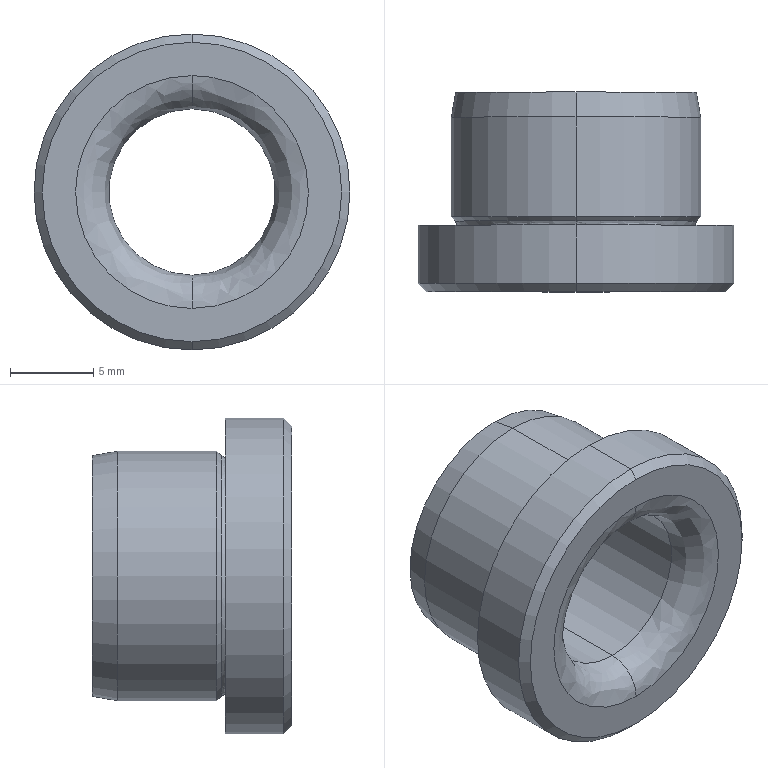Component | SolidWorks | JBH10-8-1 | 1 solid | 21 faces | box 19 x 12 x 19 mm | volume 1544 mm3 | cone 8 | cylinder 6 | spline 4 | plane 3 | commonest cylinder face diameters 10 x2 15 x2 19 x2 | material '-
STEP:
#1=COLOUR_RGB('',0.7922,0.8196,0.9333);
#2=FILL_AREA_STYLE_COLOUR('',#1);
#3=FILL_AREA_STYLE('',(#2));
#4=SURFACE_STYLE_FILL_AREA(#3);
#5=SURFACE_SIDE_STYLE('',(#4));
#6=SURFACE_STYLE_USAGE(.BOTH.,#5);
#7=PRESENTATION_STYLE_ASSIGNMENT((#6));
#8=CARTESIAN_POINT('',(-1.614,3.16,0.1969));
#9=VERTEX_POINT('',#8);
#10=CARTESIAN_POINT('',(-1.614,3.16,-0.1969));
#11=VERTEX_POINT('',#10);
#12=CARTESIAN_POINT('',(-1.614,3.16,-0.));
#13=DIRECTION('',(0.,1.,0.));
#14=DIRECTION('',(0.,0.,-1.));
#15=AXIS2_PLACEMENT_3D('',#12,#13,#14);
#16=CIRCLE('',#15,0.1969);
#17=EDGE_CURVE('',#9,#11,#16,.T.);
#18=ORIENTED_EDGE('',*,*,#17,.T.);
#19=CARTESIAN_POINT('',(-1.614,3.081,-0.2756));
#20=VERTEX_POINT('',#19);
#21=CARTESIAN_POINT('',(-1.614,3.16,-0.2756));
#22=DIRECTION('',(1.,0.,-0.));
#23=DIRECTION('',(0.,0.,-1.));
#24=AXIS2_PLACEMENT_3D('',#21,#22,#23);
#25=CIRCLE('',#24,0.07874);
#26=EDGE_CURVE('',#11,#20,#25,.T.);
#27=ORIENTED_EDGE('',*,*,#26,.T.);
#28=CARTESIAN_POINT('',(-1.614,3.081,0.2756));
#29=VERTEX_POINT('',#28);
#30=CARTESIAN_POINT('',(-1.614,3.081,-0.2756));
#31=CARTESIAN_POINT('',(-1.063,3.081,-0.2756));
#32=CARTESIAN_POINT('',(-1.063,3.081,0.2756));
#33=CARTESIAN_POINT('',(-1.614,3.081,0.2756));
#34=(BOUNDED_CURVE()B_SPLINE_CURVE(3,(#30,#31,#32,#33),.UNSPECIFIED.,.F.,.F.)B_SPLINE_CURVE_WITH_KNOTS((4,4),(0.,1.),.UNSPECIFIED.)CURVE()GEOMETRIC_REPRESENTATION_ITEM()RATIONAL_B_SPLINE_CURVE((1.,0.3333,0.3333,1.))REPRESENTATION_ITEM(''));
#35=EDGE_CURVE('',#20,#29,#34,.T.);
#36=ORIENTED_EDGE('',*,*,#35,.T.);
#37=CARTESIAN_POINT('',(-1.614,3.16,0.2756));
#38=DIRECTION('',(-1.,0.,0.));
#39=DIRECTION('',(0.,0.,1.));
#40=AXIS2_PLACEMENT_3D('',#37,#38,#39);
#41=CIRCLE('',#40,0.07874);
#42=EDGE_CURVE('',#9,#29,#41,.T.);
#43=ORIENTED_EDGE('',*,*,#42,.F.);
#44=EDGE_LOOP('',(#18,#27,#36,#43));
#45=FACE_OUTER_BOUND('',#44,.T.);
#46=CARTESIAN_POINT('',(-1.614,3.16,-0.1969));
#47=CARTESIAN_POINT('',(-1.22,3.16,-0.1969));
#48=CARTESIAN_POINT('',(-1.22,3.16,0.1969));
#49=CARTESIAN_POINT('',(-1.614,3.16,0.1969));
#50=CARTESIAN_POINT('',(-1.614,3.113,-0.1969));
#51=CARTESIAN_POINT('',(-1.22,3.113,-0.1969));
#52=CARTESIAN_POINT('',(-1.22,3.113,0.1969));
#53=CARTESIAN_POINT('',(-1.614,3.113,0.1969));
#54=CARTESIAN_POINT('',(-1.614,3.081,-0.2295));
#55=CARTESIAN_POINT('',(-1.155,3.081,-0.2295));
#56=CARTESIAN_POINT('',(-1.155,3.081,0.2295));
#57=CARTESIAN_POINT('',(-1.614,3.081,0.2295));
#58=CARTESIAN_POINT('',(-1.614,3.081,-0.2756));
#59=CARTESIAN_POINT('',(-1.063,3.081,-0.2756));
#60=CARTESIAN_POINT('',(-1.063,3.081,0.2756));
#61=CARTESIAN_POINT('',(-1.614,3.081,0.2756));
#62=(BOUNDED_SURFACE()B_SPLINE_SURFACE(3,3,((#46,#47,#48,#49),(#50,#51,#52,#53),(#54,#55,#56,#57),(#58,#59,#60,#61)),.UNSPECIFIED.,.F.,.F.,.T.)B_SPLINE_SURFACE_WITH_KNOTS((4,4),(4,4),(0.,1.),(0.,1.),.UNSPECIFIED.)GEOMETRIC_REPRESENTATION_ITEM()RATIONAL_B_SPLINE_SURFACE(((1.,0.3333,0.3333,1.),(0.8047,0.2682,0.2682,0.8047),(0.8047,0.2682,0.2682,0.8047),(1.,0.3333,0.3333,1.)))REPRESENTATION_ITEM('')SURFACE());
#63=ADVANCED_FACE('',(#45),#62,.T.);
#64=CARTESIAN_POINT('',(-1.614,3.248,-0.2854));
#65=VERTEX_POINT('',#64);
#66=CARTESIAN_POINT('',(-1.614,3.248,0.2854));
#67=VERTEX_POINT('',#66);
#68=CARTESIAN_POINT('',(-1.614,3.248,-0.));
#69=DIRECTION('',(0.,1.,0.));
#70=DIRECTION('',(-1.,0.,-0.));
#71=AXIS2_PLACEMENT_3D('',#68,#69,#70);
#72=CIRCLE('',#71,0.2854);
#73=EDGE_CURVE('',#65,#67,#72,.T.);
#74=ORIENTED_EDGE('',*,*,#73,.F.);
#75=CARTESIAN_POINT('',(-1.614,3.228,-0.3051));
#76=VERTEX_POINT('',#75);
#77=CARTESIAN_POINT('',(-1.614,3.238,-0.2953));
#78=DIRECTION('',(1.,0.,-0.));
#79=DIRECTION('',(0.,0.,-1.));
#80=AXIS2_PLACEMENT_3D('',#77,#78,#79);
#81=CIRCLE('',#80,0.01392);
#82=EDGE_CURVE('',#65,#76,#81,.T.);
#83=ORIENTED_EDGE('',*,*,#82,.T.);
#84=CARTESIAN_POINT('',(-1.614,3.228,0.3051));
#85=VERTEX_POINT('',#84);
#86=CARTESIAN_POINT('',(-1.614,3.228,-0.));
#87=DIRECTION('',(0.,-1.,0.));
#88=DIRECTION('',(0.,0.,1.));
#89=AXIS2_PLACEMENT_3D('',#86,#87,#88);
#90=CIRCLE('',#89,0.3051);
#91=EDGE_CURVE('',#85,#76,#90,.T.);
#92=ORIENTED_EDGE('',*,*,#91,.F.);
#93=CARTESIAN_POINT('',(-1.614,3.238,0.2953));
#94=DIRECTION('',(-1.,0.,0.));
#95=DIRECTION('',(0.,0.,1.));
#96=AXIS2_PLACEMENT_3D('',#93,#94,#95);
#97=CIRCLE('',#96,0.01392);
#98=EDGE_CURVE('',#67,#85,#97,.T.);
#99=ORIENTED_EDGE('',*,*,#98,.F.);
#100=EDGE_LOOP('',(#74,#83,#92,#99));
#101=FACE_OUTER_BOUND('',#100,.T.);
#102=CARTESIAN_POINT('',(-1.614,3.248,0.2854));
#103=CARTESIAN_POINT('',(-2.185,3.248,0.2854));
#104=CARTESIAN_POINT('',(-2.185,3.248,-0.2854));
#105=CARTESIAN_POINT('',(-1.614,3.248,-0.2854));
#106=CARTESIAN_POINT('',(-1.614,3.242,0.2797));
#107=CARTESIAN_POINT('',(-2.174,3.242,0.2797));
#108=CARTESIAN_POINT('',(-2.174,3.242,-0.2797));
#109=CARTESIAN_POINT('',(-1.614,3.242,-0.2797));
#110=CARTESIAN_POINT('',(-1.614,3.234,0.2797));
#111=CARTESIAN_POINT('',(-2.174,3.234,0.2797));
#112=CARTESIAN_POINT('',(-2.174,3.234,-0.2797));
#113=CARTESIAN_POINT('',(-1.614,3.234,-0.2797));
#114=CARTESIAN_POINT('',(-1.614,3.228,0.2854));
#115=CARTESIAN_POINT('',(-2.185,3.228,0.2854));
#116=CARTESIAN_POINT('',(-2.185,3.228,-0.2854));
#117=CARTESIAN_POINT('',(-1.614,3.228,-0.2854));
#118=CARTESIAN_POINT('',(-1.614,3.223,0.2912));
#119=CARTESIAN_POINT('',(-2.197,3.223,0.2912));
#120=CARTESIAN_POINT('',(-2.197,3.223,-0.2912));
#121=CARTESIAN_POINT('',(-1.614,3.223,-0.2912));
#122=CARTESIAN_POINT('',(-1.614,3.223,0.2994));
#123=CARTESIAN_POINT('',(-2.213,3.223,0.2994));
#124=CARTESIAN_POINT('',(-2.213,3.223,-0.2994));
#125=CARTESIAN_POINT('',(-1.614,3.223,-0.2994));
#126=CARTESIAN_POINT('',(-1.614,3.228,0.3051));
#127=CARTESIAN_POINT('',(-2.224,3.228,0.3051));
#128=CARTESIAN_POINT('',(-2.224,3.228,-0.3051));
#129=CARTESIAN_POINT('',(-1.614,3.228,-0.3051));
#130=(BOUNDED_SURFACE()B_SPLINE_SURFACE(3,3,((#102,#103,#104,#105),(#106,#107,#108,#109),(#110,#111,#112,#113),(#114,#115,#116,#117),(#118,#119,#120,#121),(#122,#123,#124,#125),(#126,#127,#128,#129)),.UNSPECIFIED.,.F.,.F.,.T.)B_SPLINE_SURFACE_WITH_KNOTS((4,3,4),(4,4),(0.,0.5,1.),(0.,1.),.UNSPECIFIED.)GEOMETRIC_REPRESENTATION_ITEM()RATIONAL_B_SPLINE_SURFACE(((1.,0.3333,0.3333,1.),(0.8047,0.2682,0.2682,0.8047),(0.8047,0.2682,0.2682,0.8047),(1.,0.3333,0.3333,1.),(0.8047,0.2682,0.2682,0.8047),(0.8047,0.2682,0.2682,0.8047),(1.,0.3333,0.3333,1.)))REPRESENTATION_ITEM('')SURFACE());
#131=ADVANCED_FACE('',(#101),#130,.F.);
#132=ORIENTED_EDGE('',*,*,#17,.F.);
#133=CARTESIAN_POINT('',(-1.614,3.553,0.1969));
#134=VERTEX_POINT('',#133);
#135=CARTESIAN_POINT('',(-1.614,3.356,0.1969));
#136=DIRECTION('',(0.,1.,0.));
#137=VECTOR('',#136,39.37);
#138=LINE('',#135,#137);
#139=EDGE_CURVE('',#9,#134,#138,.T.);
#140=ORIENTED_EDGE('',*,*,#139,.T.);
#141=CARTESIAN_POINT('',(-1.614,3.553,-0.1969));
#142=VERTEX_POINT('',#141);
#143=CARTESIAN_POINT('',(-1.614,3.553,-0.));
#144=DIRECTION('',(0.,-1.,0.));
#145=DIRECTION('',(0.,0.,-1.));
#146=AXIS2_PLACEMENT_3D('',#143,#144,#145);
#147=CIRCLE('',#146,0.1969);
#148=EDGE_CURVE('',#142,#134,#147,.T.);
#149=ORIENTED_EDGE('',*,*,#148,.F.);
#150=CARTESIAN_POINT('',(-1.614,3.356,-0.1969));
#151=DIRECTION('',(0.,1.,0.));
#152=VECTOR('',#151,39.37);
#153=LINE('',#150,#152);
#154=EDGE_CURVE('',#11,#142,#153,.T.);
#155=ORIENTED_EDGE('',*,*,#154,.F.);
#156=EDGE_LOOP('',(#132,#140,#149,#155));
#157=FACE_OUTER_BOUND('',#156,.T.);
#158=CARTESIAN_POINT('',(-1.614,3.356,-0.));
#159=DIRECTION('',(0.,1.,0.));
#160=DIRECTION('',(0.,0.,-1.));
#161=AXIS2_PLACEMENT_3D('',#158,#159,#160);
#162=CYLINDRICAL_SURFACE('',#161,0.1969);
#163=ADVANCED_FACE('',(#157),#162,.F.);
#164=CARTESIAN_POINT('',(-1.614,3.553,-0.2849));
#165=VERTEX_POINT('',#164);
#166=CARTESIAN_POINT('',(-1.614,3.553,0.2849));
#167=VERTEX_POINT('',#166);
#168=CARTESIAN_POINT('',(-1.614,3.553,-0.));
#169=DIRECTION('',(0.,1.,0.));
#170=DIRECTION('',(0.,0.,1.));
#171=AXIS2_PLACEMENT_3D('',#168,#169,#170);
#172=CIRCLE('',#171,0.2849);
#173=EDGE_CURVE('',#165,#167,#172,.T.);
#174=ORIENTED_EDGE('',*,*,#173,.F.);
#175=CARTESIAN_POINT('',(-1.614,3.494,-0.2953));
#176=VERTEX_POINT('',#175);
#177=CARTESIAN_POINT('',(-1.614,3.494,-0.2953));
#178=DIRECTION('',(-0.,-0.9848,-0.1736));
#179=VECTOR('',#178,39.37);
#180=LINE('',#177,#179);
#181=EDGE_CURVE('',#165,#176,#180,.T.);
#182=ORIENTED_EDGE('',*,*,#181,.T.);
#183=CARTESIAN_POINT('',(-1.614,3.494,0.2953));
#184=VERTEX_POINT('',#183);
#185=CARTESIAN_POINT('',(-1.614,3.494,-0.));
#186=DIRECTION('',(0.,1.,0.));
#187=DIRECTION('',(-1.,0.,-0.));
#188=AXIS2_PLACEMENT_3D('',#185,#186,#187);
#189=CIRCLE('',#188,0.2953);
#190=EDGE_CURVE('',#176,#184,#189,.T.);
#191=ORIENTED_EDGE('',*,*,#190,.T.);
#192=CARTESIAN_POINT('',(-1.614,3.494,0.2953));
#193=DIRECTION('',(0.,-0.9848,0.1736));
#194=VECTOR('',#193,39.37);
#195=LINE('',#192,#194);
#196=EDGE_CURVE('',#167,#184,#195,.T.);
#197=ORIENTED_EDGE('',*,*,#196,.F.);
#198=EDGE_LOOP('',(#174,#182,#191,#197));
#199=FACE_OUTER_BOUND('',#198,.T.);
#200=CARTESIAN_POINT('',(-1.614,3.494,-0.));
#201=DIRECTION('',(0.,-1.,0.));
#202=DIRECTION('',(0.,0.,1.));
#203=AXIS2_PLACEMENT_3D('',#200,#201,#202);
#204=CONICAL_SURFACE('',#203,0.2953,0.1745);
#205=ADVANCED_FACE('',(#199),#204,.T.);
#206=CARTESIAN_POINT('',(-1.614,3.258,-0.2953));
#207=VERTEX_POINT('',#206);
#208=CARTESIAN_POINT('',(-1.614,3.258,0.2953));
#209=VERTEX_POINT('',#208);
#210=CARTESIAN_POINT('',(-1.614,3.258,-0.));
#211=DIRECTION('',(0.,1.,0.));
#212=DIRECTION('',(0.,0.,-1.));
#213=AXIS2_PLACEMENT_3D('',#210,#211,#212);
#214=CIRCLE('',#213,0.2953);
#215=EDGE_CURVE('',#207,#209,#214,.T.);
#216=ORIENTED_EDGE('',*,*,#215,.T.);
#217=CARTESIAN_POINT('',(-1.614,3.376,0.2953));
#218=DIRECTION('',(0.,1.,0.));
#219=VECTOR('',#218,39.37);
#220=LINE('',#217,#219);
#221=EDGE_CURVE('',#209,#184,#220,.T.);
#222=ORIENTED_EDGE('',*,*,#221,.T.);
#223=ORIENTED_EDGE('',*,*,#190,.F.);
#224=CARTESIAN_POINT('',(-1.614,3.376,-0.2953));
#225=DIRECTION('',(0.,1.,0.));
#226=VECTOR('',#225,39.37);
#227=LINE('',#224,#226);
#228=EDGE_CURVE('',#207,#176,#227,.T.);
#229=ORIENTED_EDGE('',*,*,#228,.F.);
#230=EDGE_LOOP('',(#216,#222,#223,#229));
#231=FACE_OUTER_BOUND('',#230,.T.);
#232=CARTESIAN_POINT('',(-1.614,3.376,-0.));
#233=DIRECTION('',(0.,1.,0.));
#234=DIRECTION('',(0.,0.,-1.));
#235=AXIS2_PLACEMENT_3D('',#232,#233,#234);
#236=CYLINDRICAL_SURFACE('',#235,0.2953);
#237=ADVANCED_FACE('',(#231),#236,.T.);
#238=CARTESIAN_POINT('',(-1.614,3.081,0.3543));
#239=VERTEX_POINT('',#238);
#240=CARTESIAN_POINT('',(-1.614,3.081,-0.3543));
#241=VERTEX_POINT('',#240);
#242=CARTESIAN_POINT('',(-1.614,3.081,-0.));
#243=DIRECTION('',(0.,-1.,0.));
#244=DIRECTION('',(0.,0.,-1.));
#245=AXIS2_PLACEMENT_3D('',#242,#243,#244);
#246=CIRCLE('',#245,0.3543);
#247=EDGE_CURVE('',#239,#241,#246,.T.);
#248=ORIENTED_EDGE('',*,*,#247,.F.);
#249=CARTESIAN_POINT('',(-1.614,3.101,0.374));
#250=VERTEX_POINT('',#249);
#251=CARTESIAN_POINT('',(-1.614,3.101,0.374));
#252=DIRECTION('',(-0.,0.7071,0.7071));
#253=VECTOR('',#252,39.37);
#254=LINE('',#251,#253);
#255=EDGE_CURVE('',#239,#250,#254,.T.);
#256=ORIENTED_EDGE('',*,*,#255,.T.);
#257=CARTESIAN_POINT('',(-1.614,3.101,-0.374));
#258=VERTEX_POINT('',#257);
#259=CARTESIAN_POINT('',(-1.614,3.101,-0.));
#260=DIRECTION('',(0.,-1.,0.));
#261=DIRECTION('',(-1.,0.,-0.));
#262=AXIS2_PLACEMENT_3D('',#259,#260,#261);
#263=CIRCLE('',#262,0.374);
#264=EDGE_CURVE('',#250,#258,#263,.T.);
#265=ORIENTED_EDGE('',*,*,#264,.T.);
#266=CARTESIAN_POINT('',(-1.614,3.101,-0.374));
#267=DIRECTION('',(0.,0.7071,-0.7071));
#268=VECTOR('',#267,39.37);
#269=LINE('',#266,#268);
#270=EDGE_CURVE('',#241,#258,#269,.T.);
#271=ORIENTED_EDGE('',*,*,#270,.F.);
#272=EDGE_LOOP('',(#248,#256,#265,#271));
#273=FACE_OUTER_BOUND('',#272,.T.);
#274=CARTESIAN_POINT('',(-1.614,3.101,-0.));
#275=DIRECTION('',(0.,1.,0.));
#276=DIRECTION('',(0.,0.,-1.));
#277=AXIS2_PLACEMENT_3D('',#274,#275,#276);
#278=CONICAL_SURFACE('',#277,0.374,0.7854);
#279=ADVANCED_FACE('',(#273),#278,.T.);
#280=ORIENTED_EDGE('',*,*,#73,.T.);
#281=CARTESIAN_POINT('',(-1.614,3.258,0.2953));
#282=DIRECTION('',(-0.,0.7071,0.7071));
#283=VECTOR('',#282,39.37);
#284=LINE('',#281,#283);
#285=EDGE_CURVE('',#67,#209,#284,.T.);
#286=ORIENTED_EDGE('',*,*,#285,.T.);
#287=ORIENTED_EDGE('',*,*,#215,.F.);
#288=CARTESIAN_POINT('',(-1.614,3.258,-0.2953));
#289=DIRECTION('',(0.,0.7071,-0.7071));
#290=VECTOR('',#289,39.37);
#291=LINE('',#288,#290);
#292=EDGE_CURVE('',#65,#207,#291,.T.);
#293=ORIENTED_EDGE('',*,*,#292,.F.);
#294=EDGE_LOOP('',(#280,#286,#287,#293));
#295=FACE_OUTER_BOUND('',#294,.T.);
#296=CARTESIAN_POINT('',(-1.614,3.258,-0.));
#297=DIRECTION('',(0.,1.,0.));
#298=DIRECTION('',(0.,0.,-1.));
#299=AXIS2_PLACEMENT_3D('',#296,#297,#298);
#300=CONICAL_SURFACE('',#299,0.2953,0.7854);
#301=ADVANCED_FACE('',(#295),#300,.T.);
#302=ORIENTED_EDGE('',*,*,#264,.F.);
#303=CARTESIAN_POINT('',(-1.614,3.238,0.374));
#304=VERTEX_POINT('',#303);
#305=CARTESIAN_POINT('',(-1.614,3.169,0.374));
#306=DIRECTION('',(0.,1.,0.));
#307=VECTOR('',#306,39.37);
#308=LINE('',#305,#307);
#309=EDGE_CURVE('',#250,#304,#308,.T.);
#310=ORIENTED_EDGE('',*,*,#309,.T.);
#311=CARTESIAN_POINT('',(-1.614,3.238,-0.374));
#312=VERTEX_POINT('',#311);
#313=CARTESIAN_POINT('',(-1.614,3.238,-0.));
#314=DIRECTION('',(0.,-1.,0.));
#315=DIRECTION('',(0.,0.,-1.));
#316=AXIS2_PLACEMENT_3D('',#313,#314,#315);
#317=CIRCLE('',#316,0.374);
#318=EDGE_CURVE('',#304,#312,#317,.T.);
#319=ORIENTED_EDGE('',*,*,#318,.T.);
#320=CARTESIAN_POINT('',(-1.614,3.169,-0.374));
#321=DIRECTION('',(0.,1.,0.));
#322=VECTOR('',#321,39.37);
#323=LINE('',#320,#322);
#324=EDGE_CURVE('',#258,#312,#323,.T.);
#325=ORIENTED_EDGE('',*,*,#324,.F.);
#326=EDGE_LOOP('',(#302,#310,#319,#325));
#327=FACE_OUTER_BOUND('',#326,.T.);
#328=CARTESIAN_POINT('',(-1.614,3.169,-0.));
#329=DIRECTION('',(0.,1.,0.));
#330=DIRECTION('',(0.,0.,-1.));
#331=AXIS2_PLACEMENT_3D('',#328,#329,#330);
#332=CYLINDRICAL_SURFACE('',#331,0.374);
#333=ADVANCED_FACE('',(#327),#332,.T.);
#334=CARTESIAN_POINT('',(-1.614,3.228,-0.));
#335=DIRECTION('',(0.,-1.,0.));
#336=DIRECTION('',(0.,0.,1.));
#337=AXIS2_PLACEMENT_3D('',#334,#335,#336);
#338=CIRCLE('',#337,0.3051);
#339=EDGE_CURVE('',#76,#85,#338,.T.);
#340=ORIENTED_EDGE('',*,*,#339,.T.);
#341=CARTESIAN_POINT('',(-1.614,3.238,0.315));
#342=VERTEX_POINT('',#341);
#343=CARTESIAN_POINT('',(-1.614,3.238,0.315));
#344=DIRECTION('',(-0.,0.7071,0.7071));
#345=VECTOR('',#344,39.37);
#346=LINE('',#343,#345);
#347=EDGE_CURVE('',#85,#342,#346,.T.);
#348=ORIENTED_EDGE('',*,*,#347,.T.);
#349=CARTESIAN_POINT('',(-1.614,3.238,-0.315));
#350=VERTEX_POINT('',#349);
#351=CARTESIAN_POINT('',(-1.614,3.238,-0.));
#352=DIRECTION('',(0.,-1.,0.));
#353=DIRECTION('',(0.,0.,-1.));
#354=AXIS2_PLACEMENT_3D('',#351,#352,#353);
#355=CIRCLE('',#354,0.315);
#356=EDGE_CURVE('',#350,#342,#355,.T.);
#357=ORIENTED_EDGE('',*,*,#356,.F.);
#358=CARTESIAN_POINT('',(-1.614,3.238,-0.315));
#359=DIRECTION('',(0.,0.7071,-0.7071));
#360=VECTOR('',#359,39.37);
#361=LINE('',#358,#360);
#362=EDGE_CURVE('',#76,#350,#361,.T.);
#363=ORIENTED_EDGE('',*,*,#362,.F.);
#364=EDGE_LOOP('',(#340,#348,#357,#363));
#365=FACE_OUTER_BOUND('',#364,.T.);
#366=CARTESIAN_POINT('',(-1.614,3.238,-0.));
#367=DIRECTION('',(0.,1.,0.));
#368=DIRECTION('',(0.,0.,-1.));
#369=AXIS2_PLACEMENT_3D('',#366,#367,#368);
#370=CONICAL_SURFACE('',#369,0.315,0.7854);
#371=ADVANCED_FACE('',(#365),#370,.F.);
#372=ORIENTED_EDGE('',*,*,#139,.F.);
#373=CARTESIAN_POINT('',(-1.614,3.16,-0.));
#374=DIRECTION('',(0.,1.,0.));
#375=DIRECTION('',(0.,0.,-1.));
#376=AXIS2_PLACEMENT_3D('',#373,#374,#375);
#377=CIRCLE('',#376,0.1969);
#378=EDGE_CURVE('',#11,#9,#377,.T.);
#379=ORIENTED_EDGE('',*,*,#378,.F.);
#380=ORIENTED_EDGE('',*,*,#154,.T.);
#381=CARTESIAN_POINT('',(-1.614,3.553,-0.));
#382=DIRECTION('',(0.,-1.,0.));
#383=DIRECTION('',(0.,0.,-1.));
#384=AXIS2_PLACEMENT_3D('',#381,#382,#383);
#385=CIRCLE('',#384,0.1969);
#386=EDGE_CURVE('',#134,#142,#385,.T.);
#387=ORIENTED_EDGE('',*,*,#386,.F.);
#388=EDGE_LOOP('',(#372,#379,#380,#387));
#389=FACE_OUTER_BOUND('',#388,.T.);
#390=CARTESIAN_POINT('',(-1.614,3.356,-0.));
#391=DIRECTION('',(0.,1.,0.));
#392=DIRECTION('',(0.,0.,-1.));
#393=AXIS2_PLACEMENT_3D('',#390,#391,#392);
#394=CYLINDRICAL_SURFACE('',#393,0.1969);
#395=ADVANCED_FACE('',(#389),#394,.F.);
#396=ORIENTED_EDGE('',*,*,#148,.T.);
#397=ORIENTED_EDGE('',*,*,#386,.T.);
#398=EDGE_LOOP('',(#396,#397));
#399=FACE_BOUND('',#398,.T.);
#400=CARTESIAN_POINT('',(-1.614,3.553,-0.));
#401=DIRECTION('',(0.,1.,0.));
#402=DIRECTION('',(0.,0.,1.));
#403=AXIS2_PLACEMENT_3D('',#400,#401,#402);
#404=CIRCLE('',#403,0.2849);
#405=EDGE_CURVE('',#167,#165,#404,.T.);
#406=ORIENTED_EDGE('',*,*,#405,.T.);
#407=ORIENTED_EDGE('',*,*,#173,.T.);
#408=EDGE_LOOP('',(#406,#407));
#409=FACE_OUTER_BOUND('',#408,.T.);
#410=CARTESIAN_POINT('',(-1.855,3.553,-0.));
#411=DIRECTION('',(0.,1.,0.));
#412=DIRECTION('',(0.,0.,-1.));
#413=AXIS2_PLACEMENT_3D('',#410,#411,#412);
#414=PLANE('',#413);
#415=ADVANCED_FACE('',(#399,#409),#414,.T.);
#416=ORIENTED_EDGE('',*,*,#26,.F.);
#417=ORIENTED_EDGE('',*,*,#378,.T.);
#418=ORIENTED_EDGE('',*,*,#42,.T.);
#419=CARTESIAN_POINT('',(-1.89,3.081,-0.));
#420=VERTEX_POINT('',#419);
#421=CARTESIAN_POINT('',(-1.614,3.081,0.2756));
#422=CARTESIAN_POINT('',(-1.776,3.081,0.2756));
#423=CARTESIAN_POINT('',(-1.89,3.081,0.1614));
#424=CARTESIAN_POINT('',(-1.89,3.081,-0.));
#425=(BOUNDED_CURVE()B_SPLINE_CURVE(3,(#421,#422,#423,#424),.UNSPECIFIED.,.F.,.F.)B_SPLINE_CURVE_WITH_KNOTS((4,4),(0.,1.),.UNSPECIFIED.)CURVE()GEOMETRIC_REPRESENTATION_ITEM()RATIONAL_B_SPLINE_CURVE((1.,0.8047,0.8047,1.))REPRESENTATION_ITEM(''));
#426=EDGE_CURVE('',#29,#420,#425,.T.);
#427=ORIENTED_EDGE('',*,*,#426,.T.);
#428=CARTESIAN_POINT('',(-1.89,3.081,-0.));
#429=CARTESIAN_POINT('',(-1.89,3.081,-0.1614));
#430=CARTESIAN_POINT('',(-1.776,3.081,-0.2756));
#431=CARTESIAN_POINT('',(-1.614,3.081,-0.2756));
#432=(BOUNDED_CURVE()B_SPLINE_CURVE(3,(#428,#429,#430,#431),.UNSPECIFIED.,.F.,.F.)B_SPLINE_CURVE_WITH_KNOTS((4,4),(0.,1.),.UNSPECIFIED.)CURVE()GEOMETRIC_REPRESENTATION_ITEM()RATIONAL_B_SPLINE_CURVE((1.,0.8047,0.8047,1.))REPRESENTATION_ITEM(''));
#433=EDGE_CURVE('',#420,#20,#432,.T.);
#434=ORIENTED_EDGE('',*,*,#433,.T.);
#435=EDGE_LOOP('',(#416,#417,#418,#427,#434));
#436=FACE_OUTER_BOUND('',#435,.T.);
#437=CARTESIAN_POINT('',(-1.614,3.16,0.1969));
#438=CARTESIAN_POINT('',(-2.008,3.16,0.1969));
#439=CARTESIAN_POINT('',(-2.008,3.16,-0.1969));
#440=CARTESIAN_POINT('',(-1.614,3.16,-0.1969));
#441=CARTESIAN_POINT('',(-1.614,3.113,0.1969));
#442=CARTESIAN_POINT('',(-2.008,3.113,0.1969));
#443=CARTESIAN_POINT('',(-2.008,3.113,-0.1969));
#444=CARTESIAN_POINT('',(-1.614,3.113,-0.1969));
#445=CARTESIAN_POINT('',(-1.614,3.081,0.2295));
#446=CARTESIAN_POINT('',(-2.073,3.081,0.2295));
#447=CARTESIAN_POINT('',(-2.073,3.081,-0.2295));
#448=CARTESIAN_POINT('',(-1.614,3.081,-0.2295));
#449=CARTESIAN_POINT('',(-1.614,3.081,0.2756));
#450=CARTESIAN_POINT('',(-2.165,3.081,0.2756));
#451=CARTESIAN_POINT('',(-2.165,3.081,-0.2756));
#452=CARTESIAN_POINT('',(-1.614,3.081,-0.2756));
#453=(BOUNDED_SURFACE()B_SPLINE_SURFACE(3,3,((#437,#438,#439,#440),(#441,#442,#443,#444),(#445,#446,#447,#448),(#449,#450,#451,#452)),.UNSPECIFIED.,.F.,.F.,.T.)B_SPLINE_SURFACE_WITH_KNOTS((4,4),(4,4),(0.,1.),(0.,1.),.UNSPECIFIED.)GEOMETRIC_REPRESENTATION_ITEM()RATIONAL_B_SPLINE_SURFACE(((1.,0.3333,0.3333,1.),(0.8047,0.2682,0.2682,0.8047),(0.8047,0.2682,0.2682,0.8047),(1.,0.3333,0.3333,1.)))REPRESENTATION_ITEM('')SURFACE());
#454=ADVANCED_FACE('',(#436),#453,.T.);
#455=ORIENTED_EDGE('',*,*,#181,.F.);
#456=ORIENTED_EDGE('',*,*,#405,.F.);
#457=ORIENTED_EDGE('',*,*,#196,.T.);
#458=CARTESIAN_POINT('',(-1.614,3.494,-0.));
#459=DIRECTION('',(0.,1.,0.));
#460=DIRECTION('',(-1.,0.,-0.));
#461=AXIS2_PLACEMENT_3D('',#458,#459,#460);
#462=CIRCLE('',#461,0.2953);
#463=EDGE_CURVE('',#184,#176,#462,.T.);
#464=ORIENTED_EDGE('',*,*,#463,.T.);
#465=EDGE_LOOP('',(#455,#456,#457,#464));
#466=FACE_OUTER_BOUND('',#465,.T.);
#467=CARTESIAN_POINT('',(-1.614,3.494,-0.));
#468=DIRECTION('',(0.,-1.,0.));
#469=DIRECTION('',(0.,0.,1.));
#470=AXIS2_PLACEMENT_3D('',#467,#468,#469);
#471=CONICAL_SURFACE('',#470,0.2953,0.1745);
#472=ADVANCED_FACE('',(#466),#471,.T.);
#473=CARTESIAN_POINT('',(-1.614,3.081,-0.));
#474=DIRECTION('',(0.,-1.,0.));
#475=DIRECTION('',(0.,0.,-1.));
#476=AXIS2_PLACEMENT_3D('',#473,#474,#475);
#477=CIRCLE('',#476,0.3543);
#478=EDGE_CURVE('',#241,#239,#477,.T.);
#479=ORIENTED_EDGE('',*,*,#478,.T.);
#480=ORIENTED_EDGE('',*,*,#247,.T.);
#481=EDGE_LOOP('',(#479,#480));
#482=FACE_OUTER_BOUND('',#481,.T.);
#483=ORIENTED_EDGE('',*,*,#426,.F.);
#484=ORIENTED_EDGE('',*,*,#35,.F.);
#485=ORIENTED_EDGE('',*,*,#433,.F.);
#486=EDGE_LOOP('',(#483,#484,#485));
#487=FACE_BOUND('',#486,.T.);
#488=CARTESIAN_POINT('',(-1.929,3.081,-0.));
#489=DIRECTION('',(0.,-1.,0.));
#490=DIRECTION('',(0.,0.,1.));
#491=AXIS2_PLACEMENT_3D('',#488,#489,#490);
#492=PLANE('',#491);
#493=ADVANCED_FACE('',(#482,#487),#492,.T.);
#494=ORIENTED_EDGE('',*,*,#221,.F.);
#495=CARTESIAN_POINT('',(-1.614,3.258,-0.));
#496=DIRECTION('',(0.,1.,0.));
#497=DIRECTION('',(0.,0.,-1.));
#498=AXIS2_PLACEMENT_3D('',#495,#496,#497);
#499=CIRCLE('',#498,0.2953);
#500=EDGE_CURVE('',#209,#207,#499,.T.);
#501=ORIENTED_EDGE('',*,*,#500,.T.);
#502=ORIENTED_EDGE('',*,*,#228,.T.);
#503=ORIENTED_EDGE('',*,*,#463,.F.);
#504=EDGE_LOOP('',(#494,#501,#502,#503));
#505=FACE_OUTER_BOUND('',#504,.T.);
#506=CARTESIAN_POINT('',(-1.614,3.376,-0.));
#507=DIRECTION('',(0.,1.,0.));
#508=DIRECTION('',(0.,0.,-1.));
#509=AXIS2_PLACEMENT_3D('',#506,#507,#508);
#510=CYLINDRICAL_SURFACE('',#509,0.2953);
#511=ADVANCED_FACE('',(#505),#510,.T.);
#512=ORIENTED_EDGE('',*,*,#255,.F.);
#513=ORIENTED_EDGE('',*,*,#478,.F.);
#514=ORIENTED_EDGE('',*,*,#270,.T.);
#515=CARTESIAN_POINT('',(-1.614,3.101,-0.));
#516=DIRECTION('',(0.,-1.,0.));
#517=DIRECTION('',(-1.,0.,0.));
#518=AXIS2_PLACEMENT_3D('',#515,#516,#517);
#519=CIRCLE('',#518,0.374);
#520=EDGE_CURVE('',#258,#250,#519,.T.);
#521=ORIENTED_EDGE('',*,*,#520,.T.);
#522=EDGE_LOOP('',(#512,#513,#514,#521));
#523=FACE_OUTER_BOUND('',#522,.T.);
#524=CARTESIAN_POINT('',(-1.614,3.101,-0.));
#525=DIRECTION('',(0.,1.,0.));
#526=DIRECTION('',(0.,0.,-1.));
#527=AXIS2_PLACEMENT_3D('',#524,#525,#526);
#528=CONICAL_SURFACE('',#527,0.374,0.7854);
#529=ADVANCED_FACE('',(#523),#528,.T.);
#530=ORIENTED_EDGE('',*,*,#285,.F.);
#531=CARTESIAN_POINT('',(-1.614,3.248,-0.));
#532=DIRECTION('',(0.,1.,0.));
#533=DIRECTION('',(-1.,0.,-0.));
#534=AXIS2_PLACEMENT_3D('',#531,#532,#533);
#535=CIRCLE('',#534,0.2854);
#536=EDGE_CURVE('',#67,#65,#535,.T.);
#537=ORIENTED_EDGE('',*,*,#536,.T.);
#538=ORIENTED_EDGE('',*,*,#292,.T.);
#539=ORIENTED_EDGE('',*,*,#500,.F.);
#540=EDGE_LOOP('',(#530,#537,#538,#539));
#541=FACE_OUTER_BOUND('',#540,.T.);
#542=CARTESIAN_POINT('',(-1.614,3.258,-0.));
#543=DIRECTION('',(0.,1.,0.));
#544=DIRECTION('',(0.,0.,-1.));
#545=AXIS2_PLACEMENT_3D('',#542,#543,#544);
#546=CONICAL_SURFACE('',#545,0.2953,0.7854);
#547=ADVANCED_FACE('',(#541),#546,.T.);
#548=ORIENTED_EDGE('',*,*,#309,.F.);
#549=ORIENTED_EDGE('',*,*,#520,.F.);
#550=ORIENTED_EDGE('',*,*,#324,.T.);
#551=CARTESIAN_POINT('',(-1.614,3.238,-0.));
#552=DIRECTION('',(0.,-1.,0.));
#553=DIRECTION('',(0.,0.,-1.));
#554=AXIS2_PLACEMENT_3D('',#551,#552,#553);
#555=CIRCLE('',#554,0.374);
#556=EDGE_CURVE('',#312,#304,#555,.T.);
#557=ORIENTED_EDGE('',*,*,#556,.T.);
#558=EDGE_LOOP('',(#548,#549,#550,#557));
#559=FACE_OUTER_BOUND('',#558,.T.);
#560=CARTESIAN_POINT('',(-1.614,3.169,-0.));
#561=DIRECTION('',(0.,1.,0.));
#562=DIRECTION('',(0.,0.,-1.));
#563=AXIS2_PLACEMENT_3D('',#560,#561,#562);
#564=CYLINDRICAL_SURFACE('',#563,0.374);
#565=ADVANCED_FACE('',(#559),#564,.T.);
#566=ORIENTED_EDGE('',*,*,#82,.F.);
#567=ORIENTED_EDGE('',*,*,#536,.F.);
#568=ORIENTED_EDGE('',*,*,#98,.T.);
#569=ORIENTED_EDGE('',*,*,#339,.F.);
#570=EDGE_LOOP('',(#566,#567,#568,#569));
#571=FACE_OUTER_BOUND('',#570,.T.);
#572=CARTESIAN_POINT('',(-1.614,3.248,-0.2854));
#573=CARTESIAN_POINT('',(-1.043,3.248,-0.2854));
#574=CARTESIAN_POINT('',(-1.043,3.248,0.2854));
#575=CARTESIAN_POINT('',(-1.614,3.248,0.2854));
#576=CARTESIAN_POINT('',(-1.614,3.242,-0.2797));
#577=CARTESIAN_POINT('',(-1.055,3.242,-0.2797));
#578=CARTESIAN_POINT('',(-1.055,3.242,0.2797));
#579=CARTESIAN_POINT('',(-1.614,3.242,0.2797));
#580=CARTESIAN_POINT('',(-1.614,3.234,-0.2797));
#581=CARTESIAN_POINT('',(-1.055,3.234,-0.2797));
#582=CARTESIAN_POINT('',(-1.055,3.234,0.2797));
#583=CARTESIAN_POINT('',(-1.614,3.234,0.2797));
#584=CARTESIAN_POINT('',(-1.614,3.228,-0.2854));
#585=CARTESIAN_POINT('',(-1.043,3.228,-0.2854));
#586=CARTESIAN_POINT('',(-1.043,3.228,0.2854));
#587=CARTESIAN_POINT('',(-1.614,3.228,0.2854));
#588=CARTESIAN_POINT('',(-1.614,3.223,-0.2912));
#589=CARTESIAN_POINT('',(-1.032,3.223,-0.2912));
#590=CARTESIAN_POINT('',(-1.032,3.223,0.2912));
#591=CARTESIAN_POINT('',(-1.614,3.223,0.2912));
#592=CARTESIAN_POINT('',(-1.614,3.223,-0.2994));
#593=CARTESIAN_POINT('',(-1.015,3.223,-0.2994));
#594=CARTESIAN_POINT('',(-1.015,3.223,0.2994));
#595=CARTESIAN_POINT('',(-1.614,3.223,0.2994));
#596=CARTESIAN_POINT('',(-1.614,3.228,-0.3051));
#597=CARTESIAN_POINT('',(-1.004,3.228,-0.3051));
#598=CARTESIAN_POINT('',(-1.004,3.228,0.3051));
#599=CARTESIAN_POINT('',(-1.614,3.228,0.3051));
#600=(BOUNDED_SURFACE()B_SPLINE_SURFACE(3,3,((#572,#573,#574,#575),(#576,#577,#578,#579),(#580,#581,#582,#583),(#584,#585,#586,#587),(#588,#589,#590,#591),(#592,#593,#594,#595),(#596,#597,#598,#599)),.UNSPECIFIED.,.F.,.F.,.T.)B_SPLINE_SURFACE_WITH_KNOTS((4,3,4),(4,4),(0.,0.5,1.),(0.,1.),.UNSPECIFIED.)GEOMETRIC_REPRESENTATION_ITEM()RATIONAL_B_SPLINE_SURFACE(((1.,0.3333,0.3333,1.),(0.8047,0.2682,0.2682,0.8047),(0.8047,0.2682,0.2682,0.8047),(1.,0.3333,0.3333,1.),(0.8047,0.2682,0.2682,0.8047),(0.8047,0.2682,0.2682,0.8047),(1.,0.3333,0.3333,1.)))REPRESENTATION_ITEM('')SURFACE());
#601=ADVANCED_FACE('',(#571),#600,.F.);
#602=ORIENTED_EDGE('',*,*,#356,.T.);
#603=CARTESIAN_POINT('',(-1.614,3.238,-0.));
#604=DIRECTION('',(0.,-1.,0.));
#605=DIRECTION('',(0.,0.,-1.));
#606=AXIS2_PLACEMENT_3D('',#603,#604,#605);
#607=CIRCLE('',#606,0.315);
#608=EDGE_CURVE('',#342,#350,#607,.T.);
#609=ORIENTED_EDGE('',*,*,#608,.T.);
#610=EDGE_LOOP('',(#602,#609));
#611=FACE_BOUND('',#610,.T.);
#612=ORIENTED_EDGE('',*,*,#556,.F.);
#613=ORIENTED_EDGE('',*,*,#318,.F.);
#614=EDGE_LOOP('',(#612,#613));
#615=FACE_OUTER_BOUND('',#614,.T.);
#616=CARTESIAN_POINT('',(-1.959,3.238,-0.));
#617=DIRECTION('',(0.,1.,0.));
#618=DIRECTION('',(0.,0.,-1.));
#619=AXIS2_PLACEMENT_3D('',#616,#617,#618);
#620=PLANE('',#619);
#621=ADVANCED_FACE('',(#611,#615),#620,.T.);
#622=ORIENTED_EDGE('',*,*,#347,.F.);
#623=ORIENTED_EDGE('',*,*,#91,.T.);
#624=ORIENTED_EDGE('',*,*,#362,.T.);
#625=ORIENTED_EDGE('',*,*,#608,.F.);
#626=EDGE_LOOP('',(#622,#623,#624,#625));
#627=FACE_OUTER_BOUND('',#626,.T.);
#628=CARTESIAN_POINT('',(-1.614,3.238,-0.));
#629=DIRECTION('',(0.,1.,0.));
#630=DIRECTION('',(0.,0.,-1.));
#631=AXIS2_PLACEMENT_3D('',#628,#629,#630);
#632=CONICAL_SURFACE('',#631,0.315,0.7854);
#633=ADVANCED_FACE('',(#627),#632,.F.);
#634=CLOSED_SHELL('',(#63,#131,#163,#205,#237,#279,#301,#333,#371,#395,#415,#454,#472,#493,#511,#529,#547,#565,#601,#621,#633));
#635=MANIFOLD_SOLID_BREP('',#634);
#636=STYLED_ITEM('',(#7),#635);
#637=PRESENTATION_LAYER_ASSIGNMENT('','',(#636));
#638=(LENGTH_UNIT()NAMED_UNIT(*)SI_UNIT($,.METRE.));
#639=LENGTH_MEASURE_WITH_UNIT(LENGTH_MEASURE(0.0254),#638);
#640=DIMENSIONAL_EXPONENTS(1.,0.,0.,0.,0.,0.,0.);
#641=(CONVERSION_BASED_UNIT('',#639)LENGTH_UNIT()NAMED_UNIT(#640));
#642=UNCERTAINTY_MEASURE_WITH_UNIT(LENGTH_MEASURE(0.00001),#641,'','');
#643=(NAMED_UNIT(*)PLANE_ANGLE_UNIT()SI_UNIT($,.RADIAN.));
#644=(NAMED_UNIT(*)SI_UNIT($,.STERADIAN.)SOLID_ANGLE_UNIT());
#645=(GEOMETRIC_REPRESENTATION_CONTEXT(3)GLOBAL_UNCERTAINTY_ASSIGNED_CONTEXT((#642))GLOBAL_UNIT_ASSIGNED_CONTEXT((#641,#643,#644))REPRESENTATION_CONTEXT('',''));
#646=MECHANICAL_DESIGN_GEOMETRIC_PRESENTATION_REPRESENTATION('',(#636),#645);
#647=CARTESIAN_POINT('',(0.,0.,0.));
#648=DIRECTION('',(0.,0.,1.));
#649=DIRECTION('',(1.,0.,0.));
#650=AXIS2_PLACEMENT_3D('',#647,#648,#649);
#651=(LENGTH_UNIT()NAMED_UNIT(*)SI_UNIT($,.METRE.));
#652=LENGTH_MEASURE_WITH_UNIT(LENGTH_MEASURE(0.0254),#651);
#653=DIMENSIONAL_EXPONENTS(1.,0.,0.,0.,0.,0.,0.);
#654=(CONVERSION_BASED_UNIT('',#652)LENGTH_UNIT()NAMED_UNIT(#653));
#655=UNCERTAINTY_MEASURE_WITH_UNIT(LENGTH_MEASURE(0.00001),#654,'','');
#656=(NAMED_UNIT(*)PLANE_ANGLE_UNIT()SI_UNIT($,.RADIAN.));
#657=(NAMED_UNIT(*)SI_UNIT($,.STERADIAN.)SOLID_ANGLE_UNIT());
#658=(GEOMETRIC_REPRESENTATION_CONTEXT(3)GLOBAL_UNCERTAINTY_ASSIGNED_CONTEXT((#655))GLOBAL_UNIT_ASSIGNED_CONTEXT((#654,#656,#657))REPRESENTATION_CONTEXT('',''));
#659=ADVANCED_BREP_SHAPE_REPRESENTATION('',(#635,#650),#658);